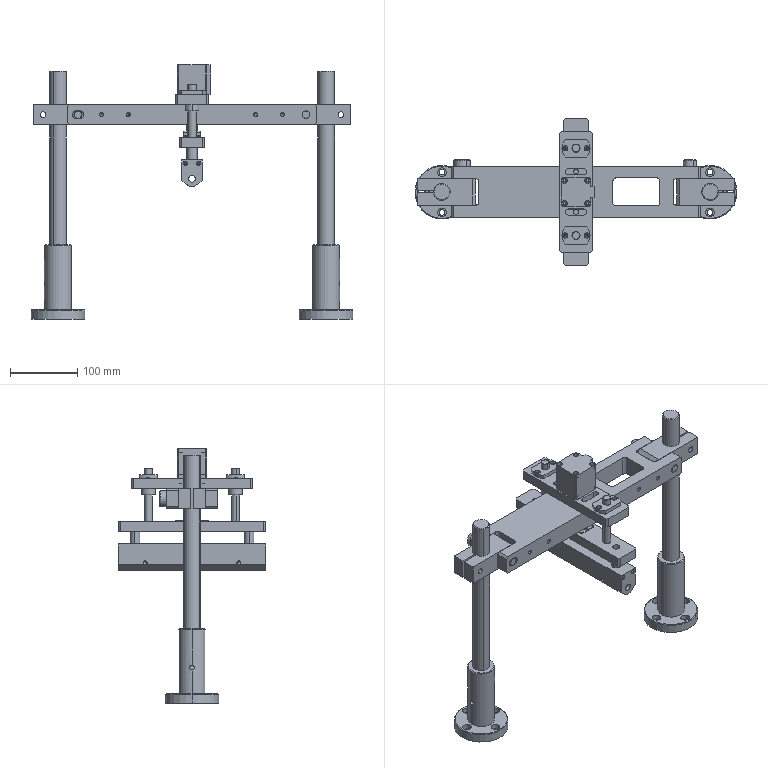Assembly | SolidWorks | mm | 21 component files | 21 solids | 645 faces | box 480 x 220 x 379.5 mm | volume 1987210 mm3 | cylinder 294 | plane 200 | cone 151 | commonest cylinder face diameters 5 x36 12 x29 8.5 x24 6.8 x22 10 x17 13 x16 11 x16 8.2 x16
Bill of materials:
CylinderFixingPlate | 1 |  | Thick rectangular plate with chamfered corners. It has three large round through-holes along its centerline, two elongated slots, four medium round holes and four small holes.
Fastener | 1 |  | Formed bracket with a hat-shaped profile and an even wall thickness. It has a raised central section, two flat flanges with one round hole each, and a U-shaped slot open to one side that cuts through the raised section.
FlangeSeat | 2 |  | Flanged tube: a round disc flange with a long hollow cylindrical stem standing on it. The flange has four through-holes on a bolt circle, and the stem has one small radial cross-hole.
GuidePost | 2 |  | Stepped cylindrical pin: a long main diameter that steps down to a shorter, smaller-diameter end.
InsulationSleeve | 2 |  | Plain hollow cylinder (tube or spacer) with one constant outside diameter and a concentric through-bore.
LMH12UULinearBearing | 2 |  | Flanged cylindrical body. The flange outline has two parallel straight edges and two convex arcs. There is a central through-bore and two smaller through-holes, one in each arc-ended lobe of the flange.
LongitudinalSealGuideShaft | 2 |  | Plain solid cylindrical rod with one constant diameter and flat ends.
LongitudinalSealMainArmFixingBracket | 2 |  | Rectangular block with one end chamfered. A large through-bore runs through the top face, and a narrow slit connects the bore to the opposite end, giving a split-clamp-like layout. Two round holes run through the block across the slit direction.
LongitudinalSealRoller | 1 |  | Long prismatic bar. Its end-face profile is a rectangle with two angled corners on one side. The end face has one round through-hole and two drilled holes with cone-shaped bottoms, and two small holes sit near the ends of one long face.
MainArm | 1 |  | Long, thick flat bar with an open slot at each end, forming a forked lug at each end. Each fork has a cross-hole through both prongs. The middle of the bar has two rectangular cutouts, the smaller one with a small hole on each side, and the long faces have several small holes.
Pin | 1 |  | Headed pin: a straight cylindrical shank with a short head of larger diameter at one end.
PinShaft | 1 |  | Headed pin: a straight cylindrical shank with a short head of larger diameter that has a chamfered outer edge.
SDA32X20 | 1 |  | Roughly square prismatic block with chamfered vertical corners and four axial through holes near the corners. A rectangular boss sticks out from one side face and has two cross holes. A short stepped round boss sticks out from one end face.
ThrustStud | 1 |  | Turned shaft or pin with three or more coaxial stepped diameters: a slender top pin, a larger middle section, and a wider collar near the base. The collar has flat cuts. Below it is a narrow groove and then a bottom flange.
TransitionPlate | 1 |  | Long flat rectangular bar or plate with chamfered corners. Six holes run along the centerline in a symmetric pattern: a larger hole near each end, a medium hole inside each of those, and two small holes near the middle.
Mates: